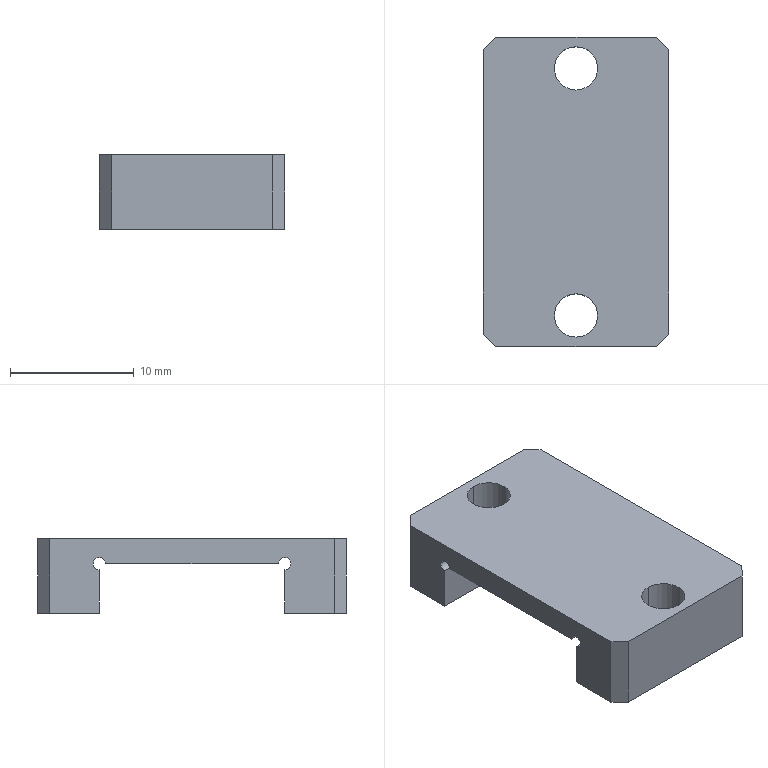Component | SolidWorks | PressurePlateA-1 | 1 solid | 21 faces | box 15 x 25 x 6 mm | volume 1205 mm3 | plane 14 | cylinder 7 | commonest cylinder face diameters 3.5 x4 1 x3
build123d program:
from build123d import *

# Parameters (mm, degrees)
SKETCH1_W                  = 25
SKETCH1_H                  = 15
EXTRUDE1_DEPTH             = 6
SKETCH2_W                  = 15
SKETCH2_H                  = 15
EXTRUDE2_DEPTH             = 4
F_3_5_3_5_DIAMETER_HOLE1_D = 3.5
CHAMFER1_SIZE              = 1
SKETCH5_R                  = 0.5
EXTRUDE3_DEPTH             = 21.427


with BuildPart() as part:
    # Sketch1 → Extrude1 (new body)
    with BuildSketch(Plane.XY):
        Rectangle(SKETCH1_W, SKETCH1_H)
    extrude(amount=EXTRUDE1_DEPTH)

    # Sketch2 → Extrude2 (cut)
    with BuildSketch(Plane.XY.offset(6)):
        Rectangle(SKETCH2_W, SKETCH2_H)
    extrude(amount=-EXTRUDE2_DEPTH, mode=Mode.SUBTRACT)

    # 3.5 _3.5_ Diameter Hole1 (through all)
    with Locations(Plane.XY.offset(6)):
        with Locations((-10, 0), (10, 0)):
            Hole(F_3_5_3_5_DIAMETER_HOLE1_D / 2)

    # Chamfer1
    chamfer1_edges = [part.edges().sort_by_distance(p)[0] for p in [
        (-12.5, 7.5, 3),
        (12.5, 7.5, 3),
        (12.5, -7.5, 3),
        (-12.5, -7.5, 3),
    ]]
    chamfer(chamfer1_edges, length=CHAMFER1_SIZE)

    # Sketch5 → Extrude3 (cut, through all)
    with BuildSketch(Plane(origin=(0, 7.5, 0), x_dir=(1, 0, 0), z_dir=(0, 1, 0))):
        with Locations((-7.5, -2)):
            Circle(SKETCH5_R)
        with Locations((7.5, -2)):
            Circle(SKETCH5_R)
    extrude(amount=-EXTRUDE3_DEPTH, mode=Mode.SUBTRACT)


solid = part.part

# Placed as in the assembly
solid = solid.moved(Location((-16.5, 0, 16), (180, 0, -90)))
STEP:
#1=CARTESIAN_POINT('',(-0.3543,0.315,0.5512));
#2=VERTEX_POINT('',#1);
#3=CARTESIAN_POINT('',(-0.3543,0.2953,0.5315));
#4=VERTEX_POINT('',#3);
#5=CARTESIAN_POINT('',(-0.3543,0.2953,0.5512));
#6=DIRECTION('',(-1.,-0.,0.));
#7=DIRECTION('',(0.,1.,0.));
#8=AXIS2_PLACEMENT_3D('',#5,#6,#7);
#9=CIRCLE('',#8,0.01969);
#10=EDGE_CURVE('',#2,#4,#9,.T.);
#11=ORIENTED_EDGE('',*,*,#10,.F.);
#12=CARTESIAN_POINT('',(-0.9449,0.315,0.5512));
#13=VERTEX_POINT('',#12);
#14=CARTESIAN_POINT('',(-0.3543,0.315,0.5512));
#15=DIRECTION('',(-1.,-0.,0.));
#16=VECTOR('',#15,39.37);
#17=LINE('',#14,#16);
#18=EDGE_CURVE('',#2,#13,#17,.T.);
#19=ORIENTED_EDGE('',*,*,#18,.T.);
#20=CARTESIAN_POINT('',(-0.9449,0.2953,0.5315));
#21=VERTEX_POINT('',#20);
#22=CARTESIAN_POINT('',(-0.9449,0.2953,0.5512));
#23=DIRECTION('',(-1.,-0.,0.));
#24=DIRECTION('',(0.,1.,0.));
#25=AXIS2_PLACEMENT_3D('',#22,#23,#24);
#26=CIRCLE('',#25,0.01969);
#27=EDGE_CURVE('',#13,#21,#26,.T.);
#28=ORIENTED_EDGE('',*,*,#27,.T.);
#29=CARTESIAN_POINT('',(-0.3543,0.2953,0.5315));
#30=DIRECTION('',(-1.,-0.,0.));
#31=VECTOR('',#30,39.37);
#32=LINE('',#29,#31);
#33=EDGE_CURVE('',#4,#21,#32,.T.);
#34=ORIENTED_EDGE('',*,*,#33,.F.);
#35=EDGE_LOOP('',(#11,#19,#28,#34));
#36=FACE_OUTER_BOUND('',#35,.T.);
#37=CARTESIAN_POINT('',(-0.3543,0.2953,0.5512));
#38=DIRECTION('',(-1.,-0.,0.));
#39=DIRECTION('',(0.,1.,0.));
#40=AXIS2_PLACEMENT_3D('',#37,#38,#39);
#41=CYLINDRICAL_SURFACE('',#40,0.01969);
#42=ADVANCED_FACE('',(#36),#41,.F.);
#43=CARTESIAN_POINT('',(-0.6496,0.4626,0.6299));
#44=VERTEX_POINT('',#43);
#45=CARTESIAN_POINT('',(-0.6496,0.3248,0.6299));
#46=VERTEX_POINT('',#45);
#47=CARTESIAN_POINT('',(-0.6496,0.3937,0.6299));
#48=DIRECTION('',(0.,0.,-1.));
#49=DIRECTION('',(0.,-1.,0.));
#50=AXIS2_PLACEMENT_3D('',#47,#48,#49);
#51=CIRCLE('',#50,0.0689);
#52=EDGE_CURVE('',#44,#46,#51,.T.);
#53=ORIENTED_EDGE('',*,*,#52,.F.);
#54=CARTESIAN_POINT('',(-0.6496,0.4626,0.3937));
#55=VERTEX_POINT('',#54);
#56=CARTESIAN_POINT('',(-0.6496,0.4626,0.3937));
#57=DIRECTION('',(0.,0.,-1.));
#58=VECTOR('',#57,39.37);
#59=LINE('',#56,#58);
#60=EDGE_CURVE('',#44,#55,#59,.T.);
#61=ORIENTED_EDGE('',*,*,#60,.T.);
#62=CARTESIAN_POINT('',(-0.6496,0.3248,0.3937));
#63=VERTEX_POINT('',#62);
#64=CARTESIAN_POINT('',(-0.6496,0.3937,0.3937));
#65=DIRECTION('',(0.,0.,-1.));
#66=DIRECTION('',(0.,-1.,0.));
#67=AXIS2_PLACEMENT_3D('',#64,#65,#66);
#68=CIRCLE('',#67,0.0689);
#69=EDGE_CURVE('',#55,#63,#68,.T.);
#70=ORIENTED_EDGE('',*,*,#69,.T.);
#71=CARTESIAN_POINT('',(-0.6496,0.3248,0.3937));
#72=DIRECTION('',(0.,0.,-1.));
#73=VECTOR('',#72,39.37);
#74=LINE('',#71,#73);
#75=EDGE_CURVE('',#46,#63,#74,.T.);
#76=ORIENTED_EDGE('',*,*,#75,.F.);
#77=EDGE_LOOP('',(#53,#61,#70,#76));
#78=FACE_OUTER_BOUND('',#77,.T.);
#79=CARTESIAN_POINT('',(-0.6496,0.3937,0.3937));
#80=DIRECTION('',(0.,0.,-1.));
#81=DIRECTION('',(0.,-1.,0.));
#82=AXIS2_PLACEMENT_3D('',#79,#80,#81);
#83=CYLINDRICAL_SURFACE('',#82,0.0689);
#84=ADVANCED_FACE('',(#78),#83,.F.);
#85=CARTESIAN_POINT('',(-0.6496,-0.3248,0.6299));
#86=VERTEX_POINT('',#85);
#87=CARTESIAN_POINT('',(-0.6496,-0.4626,0.6299));
#88=VERTEX_POINT('',#87);
#89=CARTESIAN_POINT('',(-0.6496,-0.3937,0.6299));
#90=DIRECTION('',(0.,0.,-1.));
#91=DIRECTION('',(0.,-1.,0.));
#92=AXIS2_PLACEMENT_3D('',#89,#90,#91);
#93=CIRCLE('',#92,0.0689);
#94=EDGE_CURVE('',#86,#88,#93,.T.);
#95=ORIENTED_EDGE('',*,*,#94,.F.);
#96=CARTESIAN_POINT('',(-0.6496,-0.3248,0.3937));
#97=VERTEX_POINT('',#96);
#98=CARTESIAN_POINT('',(-0.6496,-0.3248,0.3937));
#99=DIRECTION('',(0.,0.,-1.));
#100=VECTOR('',#99,39.37);
#101=LINE('',#98,#100);
#102=EDGE_CURVE('',#86,#97,#101,.T.);
#103=ORIENTED_EDGE('',*,*,#102,.T.);
#104=CARTESIAN_POINT('',(-0.6496,-0.4626,0.3937));
#105=VERTEX_POINT('',#104);
#106=CARTESIAN_POINT('',(-0.6496,-0.3937,0.3937));
#107=DIRECTION('',(0.,0.,-1.));
#108=DIRECTION('',(0.,-1.,0.));
#109=AXIS2_PLACEMENT_3D('',#106,#107,#108);
#110=CIRCLE('',#109,0.0689);
#111=EDGE_CURVE('',#97,#105,#110,.T.);
#112=ORIENTED_EDGE('',*,*,#111,.T.);
#113=CARTESIAN_POINT('',(-0.6496,-0.4626,0.3937));
#114=DIRECTION('',(0.,0.,-1.));
#115=VECTOR('',#114,39.37);
#116=LINE('',#113,#115);
#117=EDGE_CURVE('',#88,#105,#116,.T.);
#118=ORIENTED_EDGE('',*,*,#117,.F.);
#119=EDGE_LOOP('',(#95,#103,#112,#118));
#120=FACE_OUTER_BOUND('',#119,.T.);
#121=CARTESIAN_POINT('',(-0.6496,-0.3937,0.3937));
#122=DIRECTION('',(0.,0.,-1.));
#123=DIRECTION('',(0.,-1.,0.));
#124=AXIS2_PLACEMENT_3D('',#121,#122,#123);
#125=CYLINDRICAL_SURFACE('',#124,0.0689);
#126=ADVANCED_FACE('',(#120),#125,.F.);
#127=CARTESIAN_POINT('',(-0.6496,0.3937,0.3937));
#128=DIRECTION('',(0.,0.,-1.));
#129=DIRECTION('',(0.,-1.,0.));
#130=AXIS2_PLACEMENT_3D('',#127,#128,#129);
#131=CIRCLE('',#130,0.0689);
#132=EDGE_CURVE('',#63,#55,#131,.T.);
#133=ORIENTED_EDGE('',*,*,#132,.F.);
#134=ORIENTED_EDGE('',*,*,#69,.F.);
#135=EDGE_LOOP('',(#133,#134));
#136=FACE_BOUND('',#135,.T.);
#137=CARTESIAN_POINT('',(-0.9055,0.4921,0.3937));
#138=VERTEX_POINT('',#137);
#139=CARTESIAN_POINT('',(-0.3937,0.4921,0.3937));
#140=VERTEX_POINT('',#139);
#141=CARTESIAN_POINT('',(-0.3543,0.4921,0.3937));
#142=DIRECTION('',(1.,0.,0.));
#143=VECTOR('',#142,39.37);
#144=LINE('',#141,#143);
#145=EDGE_CURVE('',#138,#140,#144,.T.);
#146=ORIENTED_EDGE('',*,*,#145,.T.);
#147=CARTESIAN_POINT('',(-0.3543,0.4528,0.3937));
#148=VERTEX_POINT('',#147);
#149=CARTESIAN_POINT('',(-0.6693,0.7677,0.3937));
#150=DIRECTION('',(0.7071,-0.7071,0.));
#151=VECTOR('',#150,39.37);
#152=LINE('',#149,#151);
#153=EDGE_CURVE('',#140,#148,#152,.T.);
#154=ORIENTED_EDGE('',*,*,#153,.T.);
#155=CARTESIAN_POINT('',(-0.3543,0.2953,0.3937));
#156=VERTEX_POINT('',#155);
#157=CARTESIAN_POINT('',(-0.3543,-0.4921,0.3937));
#158=DIRECTION('',(0.,-1.,0.));
#159=VECTOR('',#158,39.37);
#160=LINE('',#157,#159);
#161=EDGE_CURVE('',#148,#156,#160,.T.);
#162=ORIENTED_EDGE('',*,*,#161,.T.);
#163=CARTESIAN_POINT('',(-0.9449,0.2953,0.3937));
#164=VERTEX_POINT('',#163);
#165=CARTESIAN_POINT('',(-0.9449,0.2953,0.3937));
#166=DIRECTION('',(1.,0.,0.));
#167=VECTOR('',#166,39.37);
#168=LINE('',#165,#167);
#169=EDGE_CURVE('',#164,#156,#168,.T.);
#170=ORIENTED_EDGE('',*,*,#169,.F.);
#171=CARTESIAN_POINT('',(-0.9449,0.4528,0.3937));
#172=VERTEX_POINT('',#171);
#173=CARTESIAN_POINT('',(-0.9449,-0.4921,0.3937));
#174=DIRECTION('',(-0.,1.,0.));
#175=VECTOR('',#174,39.37);
#176=LINE('',#173,#175);
#177=EDGE_CURVE('',#164,#172,#176,.T.);
#178=ORIENTED_EDGE('',*,*,#177,.T.);
#179=CARTESIAN_POINT('',(-0.9252,0.4724,0.3937));
#180=DIRECTION('',(0.7071,0.7071,0.));
#181=VECTOR('',#180,39.37);
#182=LINE('',#179,#181);
#183=EDGE_CURVE('',#172,#138,#182,.T.);
#184=ORIENTED_EDGE('',*,*,#183,.T.);
#185=EDGE_LOOP('',(#146,#154,#162,#170,#178,#184));
#186=FACE_OUTER_BOUND('',#185,.T.);
#187=CARTESIAN_POINT('',(-0.9449,0.4921,0.3937));
#188=DIRECTION('',(0.,0.,-1.));
#189=DIRECTION('',(0.,-1.,0.));
#190=AXIS2_PLACEMENT_3D('',#187,#188,#189);
#191=PLANE('',#190);
#192=ADVANCED_FACE('',(#136,#186),#191,.T.);
#193=CARTESIAN_POINT('',(-0.9055,0.4921,0.6299));
#194=VERTEX_POINT('',#193);
#195=CARTESIAN_POINT('',(-0.3937,0.4921,0.6299));
#196=VERTEX_POINT('',#195);
#197=CARTESIAN_POINT('',(-0.3543,0.4921,0.6299));
#198=DIRECTION('',(1.,0.,0.));
#199=VECTOR('',#198,39.37);
#200=LINE('',#197,#199);
#201=EDGE_CURVE('',#194,#196,#200,.T.);
#202=ORIENTED_EDGE('',*,*,#201,.T.);
#203=CARTESIAN_POINT('',(-0.3937,0.4921,0.3937));
#204=DIRECTION('',(0.,0.,-1.));
#205=VECTOR('',#204,39.37);
#206=LINE('',#203,#205);
#207=EDGE_CURVE('',#196,#140,#206,.T.);
#208=ORIENTED_EDGE('',*,*,#207,.T.);
#209=ORIENTED_EDGE('',*,*,#145,.F.);
#210=CARTESIAN_POINT('',(-0.9055,0.4921,0.3937));
#211=DIRECTION('',(0.,0.,1.));
#212=VECTOR('',#211,39.37);
#213=LINE('',#210,#212);
#214=EDGE_CURVE('',#138,#194,#213,.T.);
#215=ORIENTED_EDGE('',*,*,#214,.T.);
#216=EDGE_LOOP('',(#202,#208,#209,#215));
#217=FACE_OUTER_BOUND('',#216,.T.);
#218=CARTESIAN_POINT('',(-0.3543,0.4921,0.3937));
#219=DIRECTION('',(0.,-1.,0.));
#220=DIRECTION('',(0.,0.,1.));
#221=AXIS2_PLACEMENT_3D('',#218,#219,#220);
#222=PLANE('',#221);
#223=ADVANCED_FACE('',(#217),#222,.F.);
#224=CARTESIAN_POINT('',(-0.3543,-0.2953,0.5315));
#225=VERTEX_POINT('',#224);
#226=CARTESIAN_POINT('',(-0.3543,-0.2953,0.3937));
#227=VERTEX_POINT('',#226);
#228=CARTESIAN_POINT('',(-0.3543,-0.2953,0.5512));
#229=DIRECTION('',(0.,0.,-1.));
#230=VECTOR('',#229,39.37);
#231=LINE('',#228,#230);
#232=EDGE_CURVE('',#225,#227,#231,.T.);
#233=ORIENTED_EDGE('',*,*,#232,.F.);
#234=CARTESIAN_POINT('',(-0.3543,-0.2756,0.5512));
#235=VERTEX_POINT('',#234);
#236=CARTESIAN_POINT('',(-0.3543,-0.2953,0.5512));
#237=DIRECTION('',(-1.,-0.,0.));
#238=DIRECTION('',(0.,1.,0.));
#239=AXIS2_PLACEMENT_3D('',#236,#237,#238);
#240=CIRCLE('',#239,0.01969);
#241=EDGE_CURVE('',#225,#235,#240,.T.);
#242=ORIENTED_EDGE('',*,*,#241,.T.);
#243=CARTESIAN_POINT('',(-0.3543,0.2756,0.5512));
#244=VERTEX_POINT('',#243);
#245=CARTESIAN_POINT('',(-0.3543,0.2953,0.5512));
#246=DIRECTION('',(0.,-1.,0.));
#247=VECTOR('',#246,39.37);
#248=LINE('',#245,#247);
#249=EDGE_CURVE('',#244,#235,#248,.T.);
#250=ORIENTED_EDGE('',*,*,#249,.F.);
#251=CARTESIAN_POINT('',(-0.3543,0.2953,0.5512));
#252=DIRECTION('',(-1.,-0.,0.));
#253=DIRECTION('',(0.,1.,0.));
#254=AXIS2_PLACEMENT_3D('',#251,#252,#253);
#255=CIRCLE('',#254,0.01969);
#256=EDGE_CURVE('',#244,#2,#255,.T.);
#257=ORIENTED_EDGE('',*,*,#256,.T.);
#258=ORIENTED_EDGE('',*,*,#10,.T.);
#259=CARTESIAN_POINT('',(-0.3543,0.2953,0.5512));
#260=DIRECTION('',(0.,0.,-1.));
#261=VECTOR('',#260,39.37);
#262=LINE('',#259,#261);
#263=EDGE_CURVE('',#4,#156,#262,.T.);
#264=ORIENTED_EDGE('',*,*,#263,.T.);
#265=ORIENTED_EDGE('',*,*,#161,.F.);
#266=CARTESIAN_POINT('',(-0.3543,0.4528,0.6299));
#267=VERTEX_POINT('',#266);
#268=CARTESIAN_POINT('',(-0.3543,0.4528,0.3937));
#269=DIRECTION('',(0.,0.,1.));
#270=VECTOR('',#269,39.37);
#271=LINE('',#268,#270);
#272=EDGE_CURVE('',#148,#267,#271,.T.);
#273=ORIENTED_EDGE('',*,*,#272,.T.);
#274=CARTESIAN_POINT('',(-0.3543,-0.4528,0.6299));
#275=VERTEX_POINT('',#274);
#276=CARTESIAN_POINT('',(-0.3543,-0.4921,0.6299));
#277=DIRECTION('',(0.,-1.,0.));
#278=VECTOR('',#277,39.37);
#279=LINE('',#276,#278);
#280=EDGE_CURVE('',#267,#275,#279,.T.);
#281=ORIENTED_EDGE('',*,*,#280,.T.);
#282=CARTESIAN_POINT('',(-0.3543,-0.4528,0.3937));
#283=VERTEX_POINT('',#282);
#284=CARTESIAN_POINT('',(-0.3543,-0.4528,0.3937));
#285=DIRECTION('',(0.,0.,-1.));
#286=VECTOR('',#285,39.37);
#287=LINE('',#284,#286);
#288=EDGE_CURVE('',#275,#283,#287,.T.);
#289=ORIENTED_EDGE('',*,*,#288,.T.);
#290=CARTESIAN_POINT('',(-0.3543,-0.4921,0.3937));
#291=DIRECTION('',(0.,-1.,0.));
#292=VECTOR('',#291,39.37);
#293=LINE('',#290,#292);
#294=EDGE_CURVE('',#227,#283,#293,.T.);
#295=ORIENTED_EDGE('',*,*,#294,.F.);
#296=EDGE_LOOP('',(#233,#242,#250,#257,#258,#264,#265,#273,#281,#289,#295));
#297=FACE_OUTER_BOUND('',#296,.T.);
#298=CARTESIAN_POINT('',(-0.3543,-0.4921,0.3937));
#299=DIRECTION('',(-1.,-0.,0.));
#300=DIRECTION('',(-0.,1.,0.));
#301=AXIS2_PLACEMENT_3D('',#298,#299,#300);
#302=PLANE('',#301);
#303=ADVANCED_FACE('',(#297),#302,.F.);
#304=CARTESIAN_POINT('',(-0.3937,-0.4921,0.3937));
#305=VERTEX_POINT('',#304);
#306=CARTESIAN_POINT('',(-0.9055,-0.4921,0.3937));
#307=VERTEX_POINT('',#306);
#308=CARTESIAN_POINT('',(-0.3543,-0.4921,0.3937));
#309=DIRECTION('',(-1.,-0.,0.));
#310=VECTOR('',#309,39.37);
#311=LINE('',#308,#310);
#312=EDGE_CURVE('',#305,#307,#311,.T.);
#313=ORIENTED_EDGE('',*,*,#312,.F.);
#314=CARTESIAN_POINT('',(-0.3937,-0.4921,0.6299));
#315=VERTEX_POINT('',#314);
#316=CARTESIAN_POINT('',(-0.3937,-0.4921,0.3937));
#317=DIRECTION('',(0.,0.,1.));
#318=VECTOR('',#317,39.37);
#319=LINE('',#316,#318);
#320=EDGE_CURVE('',#305,#315,#319,.T.);
#321=ORIENTED_EDGE('',*,*,#320,.T.);
#322=CARTESIAN_POINT('',(-0.9055,-0.4921,0.6299));
#323=VERTEX_POINT('',#322);
#324=CARTESIAN_POINT('',(-0.3543,-0.4921,0.6299));
#325=DIRECTION('',(-1.,-0.,0.));
#326=VECTOR('',#325,39.37);
#327=LINE('',#324,#326);
#328=EDGE_CURVE('',#315,#323,#327,.T.);
#329=ORIENTED_EDGE('',*,*,#328,.T.);
#330=CARTESIAN_POINT('',(-0.9055,-0.4921,0.3937));
#331=DIRECTION('',(0.,0.,-1.));
#332=VECTOR('',#331,39.37);
#333=LINE('',#330,#332);
#334=EDGE_CURVE('',#323,#307,#333,.T.);
#335=ORIENTED_EDGE('',*,*,#334,.T.);
#336=EDGE_LOOP('',(#313,#321,#329,#335));
#337=FACE_OUTER_BOUND('',#336,.T.);
#338=CARTESIAN_POINT('',(-0.3543,-0.4921,0.3937));
#339=DIRECTION('',(-0.,1.,0.));
#340=DIRECTION('',(0.,0.,-1.));
#341=AXIS2_PLACEMENT_3D('',#338,#339,#340);
#342=PLANE('',#341);
#343=ADVANCED_FACE('',(#337),#342,.F.);
#344=CARTESIAN_POINT('',(-0.9449,-0.2756,0.5512));
#345=VERTEX_POINT('',#344);
#346=CARTESIAN_POINT('',(-0.9449,0.2756,0.5512));
#347=VERTEX_POINT('',#346);
#348=CARTESIAN_POINT('',(-0.9449,0.2953,0.5512));
#349=DIRECTION('',(-0.,1.,0.));
#350=VECTOR('',#349,39.37);
#351=LINE('',#348,#350);
#352=EDGE_CURVE('',#345,#347,#351,.T.);
#353=ORIENTED_EDGE('',*,*,#352,.F.);
#354=CARTESIAN_POINT('',(-0.9449,-0.2953,0.5315));
#355=VERTEX_POINT('',#354);
#356=CARTESIAN_POINT('',(-0.9449,-0.2953,0.5512));
#357=DIRECTION('',(-1.,-0.,0.));
#358=DIRECTION('',(0.,1.,0.));
#359=AXIS2_PLACEMENT_3D('',#356,#357,#358);
#360=CIRCLE('',#359,0.01969);
#361=EDGE_CURVE('',#355,#345,#360,.T.);
#362=ORIENTED_EDGE('',*,*,#361,.F.);
#363=CARTESIAN_POINT('',(-0.9449,-0.2953,0.3937));
#364=VERTEX_POINT('',#363);
#365=CARTESIAN_POINT('',(-0.9449,-0.2953,0.5512));
#366=DIRECTION('',(0.,0.,-1.));
#367=VECTOR('',#366,39.37);
#368=LINE('',#365,#367);
#369=EDGE_CURVE('',#355,#364,#368,.T.);
#370=ORIENTED_EDGE('',*,*,#369,.T.);
#371=CARTESIAN_POINT('',(-0.9449,-0.4528,0.3937));
#372=VERTEX_POINT('',#371);
#373=CARTESIAN_POINT('',(-0.9449,-0.4921,0.3937));
#374=DIRECTION('',(-0.,1.,0.));
#375=VECTOR('',#374,39.37);
#376=LINE('',#373,#375);
#377=EDGE_CURVE('',#372,#364,#376,.T.);
#378=ORIENTED_EDGE('',*,*,#377,.F.);
#379=CARTESIAN_POINT('',(-0.9449,-0.4528,0.6299));
#380=VERTEX_POINT('',#379);
#381=CARTESIAN_POINT('',(-0.9449,-0.4528,0.3937));
#382=DIRECTION('',(0.,0.,1.));
#383=VECTOR('',#382,39.37);
#384=LINE('',#381,#383);
#385=EDGE_CURVE('',#372,#380,#384,.T.);
#386=ORIENTED_EDGE('',*,*,#385,.T.);
#387=CARTESIAN_POINT('',(-0.9449,0.4528,0.6299));
#388=VERTEX_POINT('',#387);
#389=CARTESIAN_POINT('',(-0.9449,-0.4921,0.6299));
#390=DIRECTION('',(-0.,1.,0.));
#391=VECTOR('',#390,39.37);
#392=LINE('',#389,#391);
#393=EDGE_CURVE('',#380,#388,#392,.T.);
#394=ORIENTED_EDGE('',*,*,#393,.T.);
#395=CARTESIAN_POINT('',(-0.9449,0.4528,0.3937));
#396=DIRECTION('',(0.,0.,-1.));
#397=VECTOR('',#396,39.37);
#398=LINE('',#395,#397);
#399=EDGE_CURVE('',#388,#172,#398,.T.);
#400=ORIENTED_EDGE('',*,*,#399,.T.);
#401=ORIENTED_EDGE('',*,*,#177,.F.);
#402=CARTESIAN_POINT('',(-0.9449,0.2953,0.5512));
#403=DIRECTION('',(0.,0.,-1.));
#404=VECTOR('',#403,39.37);
#405=LINE('',#402,#404);
#406=EDGE_CURVE('',#21,#164,#405,.T.);
#407=ORIENTED_EDGE('',*,*,#406,.F.);
#408=ORIENTED_EDGE('',*,*,#27,.F.);
#409=CARTESIAN_POINT('',(-0.9449,0.2953,0.5512));
#410=DIRECTION('',(-1.,-0.,0.));
#411=DIRECTION('',(0.,1.,0.));
#412=AXIS2_PLACEMENT_3D('',#409,#410,#411);
#413=CIRCLE('',#412,0.01969);
#414=EDGE_CURVE('',#347,#13,#413,.T.);
#415=ORIENTED_EDGE('',*,*,#414,.F.);
#416=EDGE_LOOP('',(#353,#362,#370,#378,#386,#394,#400,#401,#407,#408,#415));
#417=FACE_OUTER_BOUND('',#416,.T.);
#418=CARTESIAN_POINT('',(-0.9449,-0.4921,0.3937));
#419=DIRECTION('',(1.,0.,0.));
#420=DIRECTION('',(0.,-1.,0.));
#421=AXIS2_PLACEMENT_3D('',#418,#419,#420);
#422=PLANE('',#421);
#423=ADVANCED_FACE('',(#417),#422,.F.);
#424=CARTESIAN_POINT('',(-0.6496,-0.3937,0.3937));
#425=DIRECTION('',(0.,0.,-1.));
#426=DIRECTION('',(0.,-1.,0.));
#427=AXIS2_PLACEMENT_3D('',#424,#425,#426);
#428=CIRCLE('',#427,0.0689);
#429=EDGE_CURVE('',#105,#97,#428,.T.);
#430=ORIENTED_EDGE('',*,*,#429,.F.);
#431=ORIENTED_EDGE('',*,*,#111,.F.);
#432=EDGE_LOOP('',(#430,#431));
#433=FACE_BOUND('',#432,.T.);
#434=ORIENTED_EDGE('',*,*,#294,.T.);
#435=CARTESIAN_POINT('',(-0.1772,-0.2756,0.3937));
#436=DIRECTION('',(-0.7071,-0.7071,0.));
#437=VECTOR('',#436,39.37);
#438=LINE('',#435,#437);
#439=EDGE_CURVE('',#283,#305,#438,.T.);
#440=ORIENTED_EDGE('',*,*,#439,.T.);
#441=ORIENTED_EDGE('',*,*,#312,.T.);
#442=CARTESIAN_POINT('',(-1.417,0.01969,0.3937));
#443=DIRECTION('',(-0.7071,0.7071,0.));
#444=VECTOR('',#443,39.37);
#445=LINE('',#442,#444);
#446=EDGE_CURVE('',#307,#372,#445,.T.);
#447=ORIENTED_EDGE('',*,*,#446,.T.);
#448=ORIENTED_EDGE('',*,*,#377,.T.);
#449=CARTESIAN_POINT('',(-0.9449,-0.2953,0.3937));
#450=DIRECTION('',(-1.,-0.,0.));
#451=VECTOR('',#450,39.37);
#452=LINE('',#449,#451);
#453=EDGE_CURVE('',#227,#364,#452,.T.);
#454=ORIENTED_EDGE('',*,*,#453,.F.);
#455=EDGE_LOOP('',(#434,#440,#441,#447,#448,#454));
#456=FACE_OUTER_BOUND('',#455,.T.);
#457=CARTESIAN_POINT('',(-0.9449,0.4921,0.3937));
#458=DIRECTION('',(0.,0.,-1.));
#459=DIRECTION('',(0.,-1.,0.));
#460=AXIS2_PLACEMENT_3D('',#457,#458,#459);
#461=PLANE('',#460);
#462=ADVANCED_FACE('',(#433,#456),#461,.T.);
#463=CARTESIAN_POINT('',(-0.6496,0.3937,0.6299));
#464=DIRECTION('',(0.,0.,-1.));
#465=DIRECTION('',(0.,-1.,0.));
#466=AXIS2_PLACEMENT_3D('',#463,#464,#465);
#467=CIRCLE('',#466,0.0689);
#468=EDGE_CURVE('',#46,#44,#467,.T.);
#469=ORIENTED_EDGE('',*,*,#468,.T.);
#470=ORIENTED_EDGE('',*,*,#52,.T.);
#471=EDGE_LOOP('',(#469,#470));
#472=FACE_BOUND('',#471,.T.);
#473=CARTESIAN_POINT('',(-0.6496,-0.3937,0.6299));
#474=DIRECTION('',(0.,0.,-1.));
#475=DIRECTION('',(0.,-1.,0.));
#476=AXIS2_PLACEMENT_3D('',#473,#474,#475);
#477=CIRCLE('',#476,0.0689);
#478=EDGE_CURVE('',#88,#86,#477,.T.);
#479=ORIENTED_EDGE('',*,*,#478,.T.);
#480=ORIENTED_EDGE('',*,*,#94,.T.);
#481=EDGE_LOOP('',(#479,#480));
#482=FACE_BOUND('',#481,.T.);
#483=ORIENTED_EDGE('',*,*,#328,.F.);
#484=CARTESIAN_POINT('',(-0.3937,-0.4921,0.6299));
#485=DIRECTION('',(0.7071,0.7071,0.));
#486=VECTOR('',#485,39.37);
#487=LINE('',#484,#486);
#488=EDGE_CURVE('',#315,#275,#487,.T.);
#489=ORIENTED_EDGE('',*,*,#488,.T.);
#490=ORIENTED_EDGE('',*,*,#280,.F.);
#491=CARTESIAN_POINT('',(-0.3543,0.4528,0.6299));
#492=DIRECTION('',(-0.7071,0.7071,0.));
#493=VECTOR('',#492,39.37);
#494=LINE('',#491,#493);
#495=EDGE_CURVE('',#267,#196,#494,.T.);
#496=ORIENTED_EDGE('',*,*,#495,.T.);
#497=ORIENTED_EDGE('',*,*,#201,.F.);
#498=CARTESIAN_POINT('',(-0.9055,0.4921,0.6299));
#499=DIRECTION('',(-0.7071,-0.7071,0.));
#500=VECTOR('',#499,39.37);
#501=LINE('',#498,#500);
#502=EDGE_CURVE('',#194,#388,#501,.T.);
#503=ORIENTED_EDGE('',*,*,#502,.T.);
#504=ORIENTED_EDGE('',*,*,#393,.F.);
#505=CARTESIAN_POINT('',(-0.9449,-0.4528,0.6299));
#506=DIRECTION('',(0.7071,-0.7071,0.));
#507=VECTOR('',#506,39.37);
#508=LINE('',#505,#507);
#509=EDGE_CURVE('',#380,#323,#508,.T.);
#510=ORIENTED_EDGE('',*,*,#509,.T.);
#511=EDGE_LOOP('',(#483,#489,#490,#496,#497,#503,#504,#510));
#512=FACE_OUTER_BOUND('',#511,.T.);
#513=CARTESIAN_POINT('',(-0.9449,0.4921,0.6299));
#514=DIRECTION('',(0.,0.,-1.));
#515=DIRECTION('',(0.,-1.,0.));
#516=AXIS2_PLACEMENT_3D('',#513,#514,#515);
#517=PLANE('',#516);
#518=ADVANCED_FACE('',(#472,#482,#512),#517,.F.);
#519=ORIENTED_EDGE('',*,*,#263,.F.);
#520=ORIENTED_EDGE('',*,*,#33,.T.);
#521=ORIENTED_EDGE('',*,*,#406,.T.);
#522=ORIENTED_EDGE('',*,*,#169,.T.);
#523=EDGE_LOOP('',(#519,#520,#521,#522));
#524=FACE_OUTER_BOUND('',#523,.T.);
#525=CARTESIAN_POINT('',(-0.9449,0.2953,0.5512));
#526=DIRECTION('',(-0.,1.,0.));
#527=DIRECTION('',(1.,0.,0.));
#528=AXIS2_PLACEMENT_3D('',#525,#526,#527);
#529=PLANE('',#528);
#530=ADVANCED_FACE('',(#524),#529,.F.);
#531=ORIENTED_EDGE('',*,*,#369,.F.);
#532=CARTESIAN_POINT('',(-0.3543,-0.2953,0.5315));
#533=DIRECTION('',(1.,0.,0.));
#534=VECTOR('',#533,39.37);
#535=LINE('',#532,#534);
#536=EDGE_CURVE('',#355,#225,#535,.T.);
#537=ORIENTED_EDGE('',*,*,#536,.T.);
#538=ORIENTED_EDGE('',*,*,#232,.T.);
#539=ORIENTED_EDGE('',*,*,#453,.T.);
#540=EDGE_LOOP('',(#531,#537,#538,#539));
#541=FACE_OUTER_BOUND('',#540,.T.);
#542=CARTESIAN_POINT('',(-0.9449,-0.2953,0.5512));
#543=DIRECTION('',(0.,-1.,0.));
#544=DIRECTION('',(-1.,-0.,0.));
#545=AXIS2_PLACEMENT_3D('',#542,#543,#544);
#546=PLANE('',#545);
#547=ADVANCED_FACE('',(#541),#546,.F.);
#548=CARTESIAN_POINT('',(-0.3543,-0.2756,0.5512));
#549=DIRECTION('',(1.,0.,0.));
#550=VECTOR('',#549,39.37);
#551=LINE('',#548,#550);
#552=EDGE_CURVE('',#345,#235,#551,.T.);
#553=ORIENTED_EDGE('',*,*,#552,.F.);
#554=ORIENTED_EDGE('',*,*,#352,.T.);
#555=CARTESIAN_POINT('',(-0.3543,0.2756,0.5512));
#556=DIRECTION('',(-1.,-0.,0.));
#557=VECTOR('',#556,39.37);
#558=LINE('',#555,#557);
#559=EDGE_CURVE('',#244,#347,#558,.T.);
#560=ORIENTED_EDGE('',*,*,#559,.F.);
#561=ORIENTED_EDGE('',*,*,#249,.T.);
#562=EDGE_LOOP('',(#553,#554,#560,#561));
#563=FACE_OUTER_BOUND('',#562,.T.);
#564=CARTESIAN_POINT('',(-0.3543,0.2953,0.5512));
#565=DIRECTION('',(0.,0.,-1.));
#566=DIRECTION('',(0.,-1.,0.));
#567=AXIS2_PLACEMENT_3D('',#564,#565,#566);
#568=PLANE('',#567);
#569=ADVANCED_FACE('',(#563),#568,.T.);
#570=ORIENTED_EDGE('',*,*,#102,.F.);
#571=ORIENTED_EDGE('',*,*,#478,.F.);
#572=ORIENTED_EDGE('',*,*,#117,.T.);
#573=ORIENTED_EDGE('',*,*,#429,.T.);
#574=EDGE_LOOP('',(#570,#571,#572,#573));
#575=FACE_OUTER_BOUND('',#574,.T.);
#576=CARTESIAN_POINT('',(-0.6496,-0.3937,0.3937));
#577=DIRECTION('',(0.,0.,-1.));
#578=DIRECTION('',(0.,-1.,0.));
#579=AXIS2_PLACEMENT_3D('',#576,#577,#578);
#580=CYLINDRICAL_SURFACE('',#579,0.0689);
#581=ADVANCED_FACE('',(#575),#580,.F.);
#582=ORIENTED_EDGE('',*,*,#60,.F.);
#583=ORIENTED_EDGE('',*,*,#468,.F.);
#584=ORIENTED_EDGE('',*,*,#75,.T.);
#585=ORIENTED_EDGE('',*,*,#132,.T.);
#586=EDGE_LOOP('',(#582,#583,#584,#585));
#587=FACE_OUTER_BOUND('',#586,.T.);
#588=CARTESIAN_POINT('',(-0.6496,0.3937,0.3937));
#589=DIRECTION('',(0.,0.,-1.));
#590=DIRECTION('',(0.,-1.,0.));
#591=AXIS2_PLACEMENT_3D('',#588,#589,#590);
#592=CYLINDRICAL_SURFACE('',#591,0.0689);
#593=ADVANCED_FACE('',(#587),#592,.F.);
#594=ORIENTED_EDGE('',*,*,#439,.F.);
#595=ORIENTED_EDGE('',*,*,#288,.F.);
#596=ORIENTED_EDGE('',*,*,#488,.F.);
#597=ORIENTED_EDGE('',*,*,#320,.F.);
#598=EDGE_LOOP('',(#594,#595,#596,#597));
#599=FACE_OUTER_BOUND('',#598,.T.);
#600=CARTESIAN_POINT('',(-0.3937,-0.4921,0.3937));
#601=DIRECTION('',(-0.7071,0.7071,0.));
#602=DIRECTION('',(0.7071,0.7071,0.));
#603=AXIS2_PLACEMENT_3D('',#600,#601,#602);
#604=PLANE('',#603);
#605=ADVANCED_FACE('',(#599),#604,.F.);
#606=ORIENTED_EDGE('',*,*,#153,.F.);
#607=ORIENTED_EDGE('',*,*,#207,.F.);
#608=ORIENTED_EDGE('',*,*,#495,.F.);
#609=ORIENTED_EDGE('',*,*,#272,.F.);
#610=EDGE_LOOP('',(#606,#607,#608,#609));
#611=FACE_OUTER_BOUND('',#610,.T.);
#612=CARTESIAN_POINT('',(-0.3543,0.4528,0.3937));
#613=DIRECTION('',(-0.7071,-0.7071,0.));
#614=DIRECTION('',(-0.7071,0.7071,0.));
#615=AXIS2_PLACEMENT_3D('',#612,#613,#614);
#616=PLANE('',#615);
#617=ADVANCED_FACE('',(#611),#616,.F.);
#618=ORIENTED_EDGE('',*,*,#446,.F.);
#619=ORIENTED_EDGE('',*,*,#334,.F.);
#620=ORIENTED_EDGE('',*,*,#509,.F.);
#621=ORIENTED_EDGE('',*,*,#385,.F.);
#622=EDGE_LOOP('',(#618,#619,#620,#621));
#623=FACE_OUTER_BOUND('',#622,.T.);
#624=CARTESIAN_POINT('',(-0.9449,-0.4528,0.3937));
#625=DIRECTION('',(0.7071,0.7071,0.));
#626=DIRECTION('',(0.7071,-0.7071,0.));
#627=AXIS2_PLACEMENT_3D('',#624,#625,#626);
#628=PLANE('',#627);
#629=ADVANCED_FACE('',(#623),#628,.F.);
#630=ORIENTED_EDGE('',*,*,#183,.F.);
#631=ORIENTED_EDGE('',*,*,#399,.F.);
#632=ORIENTED_EDGE('',*,*,#502,.F.);
#633=ORIENTED_EDGE('',*,*,#214,.F.);
#634=EDGE_LOOP('',(#630,#631,#632,#633));
#635=FACE_OUTER_BOUND('',#634,.T.);
#636=CARTESIAN_POINT('',(-0.9055,0.4921,0.3937));
#637=DIRECTION('',(0.7071,-0.7071,0.));
#638=DIRECTION('',(-0.7071,-0.7071,0.));
#639=AXIS2_PLACEMENT_3D('',#636,#637,#638);
#640=PLANE('',#639);
#641=ADVANCED_FACE('',(#635),#640,.F.);
#642=ORIENTED_EDGE('',*,*,#18,.F.);
#643=ORIENTED_EDGE('',*,*,#256,.F.);
#644=ORIENTED_EDGE('',*,*,#559,.T.);
#645=ORIENTED_EDGE('',*,*,#414,.T.);
#646=EDGE_LOOP('',(#642,#643,#644,#645));
#647=FACE_OUTER_BOUND('',#646,.T.);
#648=CARTESIAN_POINT('',(-0.3543,0.2953,0.5512));
#649=DIRECTION('',(-1.,-0.,0.));
#650=DIRECTION('',(0.,1.,0.));
#651=AXIS2_PLACEMENT_3D('',#648,#649,#650);
#652=CYLINDRICAL_SURFACE('',#651,0.01969);
#653=ADVANCED_FACE('',(#647),#652,.F.);
#654=ORIENTED_EDGE('',*,*,#361,.T.);
#655=ORIENTED_EDGE('',*,*,#552,.T.);
#656=ORIENTED_EDGE('',*,*,#241,.F.);
#657=ORIENTED_EDGE('',*,*,#536,.F.);
#658=EDGE_LOOP('',(#654,#655,#656,#657));
#659=FACE_OUTER_BOUND('',#658,.T.);
#660=CARTESIAN_POINT('',(-0.3543,-0.2953,0.5512));
#661=DIRECTION('',(-1.,-0.,0.));
#662=DIRECTION('',(0.,1.,0.));
#663=AXIS2_PLACEMENT_3D('',#660,#661,#662);
#664=CYLINDRICAL_SURFACE('',#663,0.01969);
#665=ADVANCED_FACE('',(#659),#664,.F.);
#666=CLOSED_SHELL('',(#42,#84,#126,#192,#223,#303,#343,#423,#462,#518,#530,#547,#569,#581,#593,#605,#617,#629,#641,#653,#665));
#667=MANIFOLD_SOLID_BREP('',#666);
#668=CARTESIAN_POINT('',(0.,0.,0.));
#669=DIRECTION('',(0.,0.,1.));
#670=DIRECTION('',(1.,0.,0.));
#671=AXIS2_PLACEMENT_3D('',#668,#669,#670);
#672=(LENGTH_UNIT()NAMED_UNIT(*)SI_UNIT($,.METRE.));
#673=LENGTH_MEASURE_WITH_UNIT(LENGTH_MEASURE(0.0254),#672);
#674=DIMENSIONAL_EXPONENTS(1.,0.,0.,0.,0.,0.,0.);
#675=(CONVERSION_BASED_UNIT('',#673)LENGTH_UNIT()NAMED_UNIT(#674));
#676=UNCERTAINTY_MEASURE_WITH_UNIT(LENGTH_MEASURE(0.00001),#675,'','');
#677=(NAMED_UNIT(*)PLANE_ANGLE_UNIT()SI_UNIT($,.RADIAN.));
#678=(NAMED_UNIT(*)SI_UNIT($,.STERADIAN.)SOLID_ANGLE_UNIT());
#679=(GEOMETRIC_REPRESENTATION_CONTEXT(3)GLOBAL_UNCERTAINTY_ASSIGNED_CONTEXT((#676))GLOBAL_UNIT_ASSIGNED_CONTEXT((#675,#677,#678))REPRESENTATION_CONTEXT('',''));
#680=ADVANCED_BREP_SHAPE_REPRESENTATION('',(#667,#671),#679);
#681=COLOUR_RGB('',0.7922,0.8196,0.9333);
#682=FILL_AREA_STYLE_COLOUR('',#681);
#683=FILL_AREA_STYLE('',(#682));
#684=SURFACE_STYLE_FILL_AREA(#683);
#685=SURFACE_SIDE_STYLE('',(#684));
#686=SURFACE_STYLE_USAGE(.BOTH.,#685);
#687=PRESENTATION_STYLE_ASSIGNMENT((#686));
#688=STYLED_ITEM('',(#687),#667);
#689=(LENGTH_UNIT()NAMED_UNIT(*)SI_UNIT($,.METRE.));
#690=LENGTH_MEASURE_WITH_UNIT(LENGTH_MEASURE(0.0254),#689);
#691=DIMENSIONAL_EXPONENTS(1.,0.,0.,0.,0.,0.,0.);
#692=(CONVERSION_BASED_UNIT('',#690)LENGTH_UNIT()NAMED_UNIT(#691));
#693=UNCERTAINTY_MEASURE_WITH_UNIT(LENGTH_MEASURE(0.00001),#692,'','');
#694=(NAMED_UNIT(*)PLANE_ANGLE_UNIT()SI_UNIT($,.RADIAN.));
#695=(NAMED_UNIT(*)SI_UNIT($,.STERADIAN.)SOLID_ANGLE_UNIT());
#696=(GEOMETRIC_REPRESENTATION_CONTEXT(3)GLOBAL_UNCERTAINTY_ASSIGNED_CONTEXT((#693))GLOBAL_UNIT_ASSIGNED_CONTEXT((#692,#694,#695))REPRESENTATION_CONTEXT('',''));
#697=MECHANICAL_DESIGN_GEOMETRIC_PRESENTATION_REPRESENTATION('',(#688),#696);
#698=PRESENTATION_LAYER_ASSIGNMENT('','',(#688));